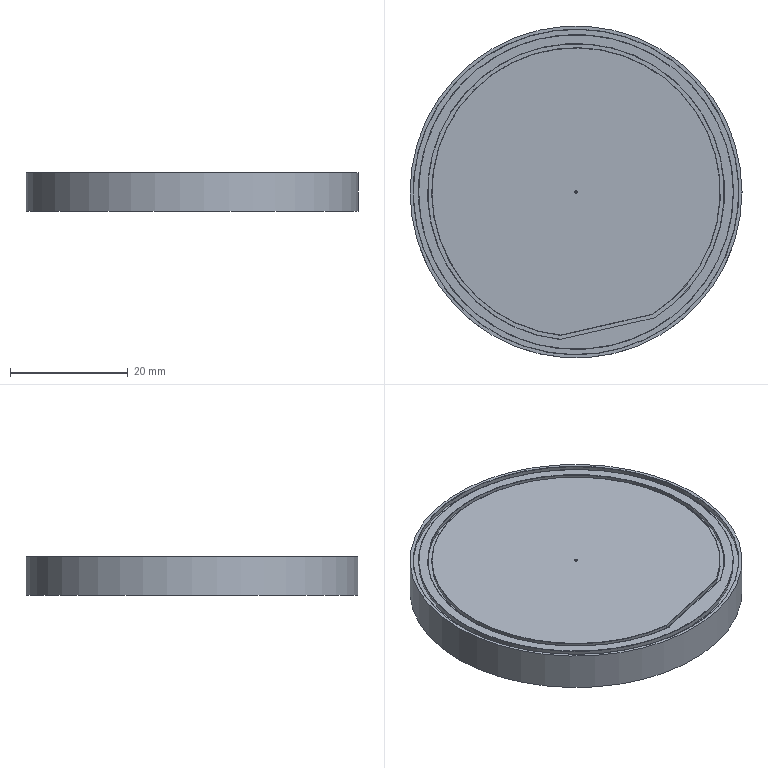CAM job | NX | mm | 3-axis | 1 set-up | 4 operations | part box 56.4 x 56.4 x 6.54
set-up 1
1. Z-Level Milling | Mill Mill5 D0.5 | ZLEVEL_PROFILE | path 15527.93 mm | 6.16 min
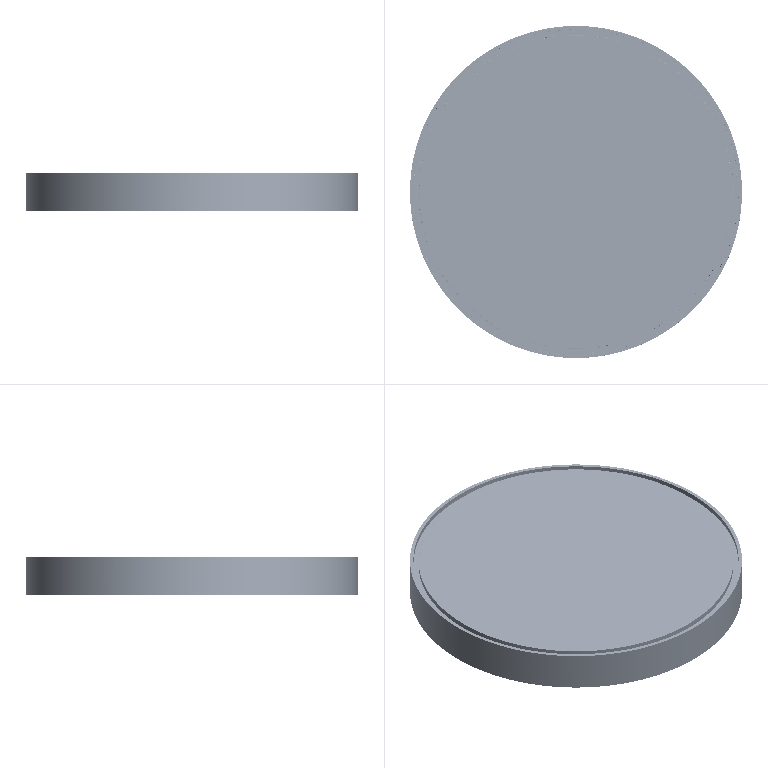2. Z-Level Milling | Mill Mill5 D0.5 | ZLEVEL_PROFILE_COPY | path 11539.132 mm | 4.583 min
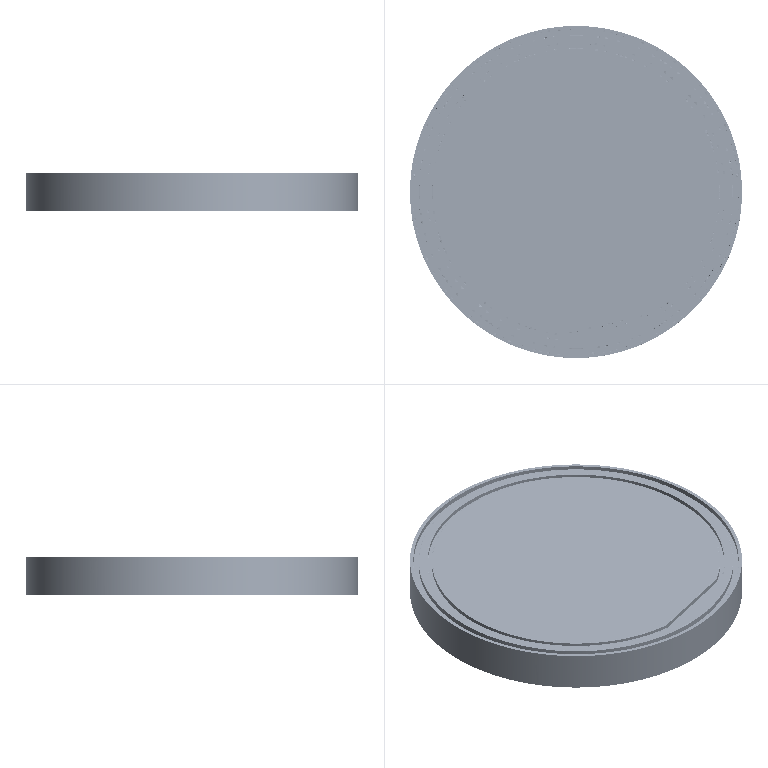3. Z-Level Milling | Mill Mill5 D0.5 | ZLEVEL_PROFILE_COPY_1 | path 15527.93 mm | 6.16 min
4. Z-Level Milling | Mill Mill5 D0.5 | ZLEVEL_PROFILE_COPY_COPY | path 11539.132 mm | 4.583 min